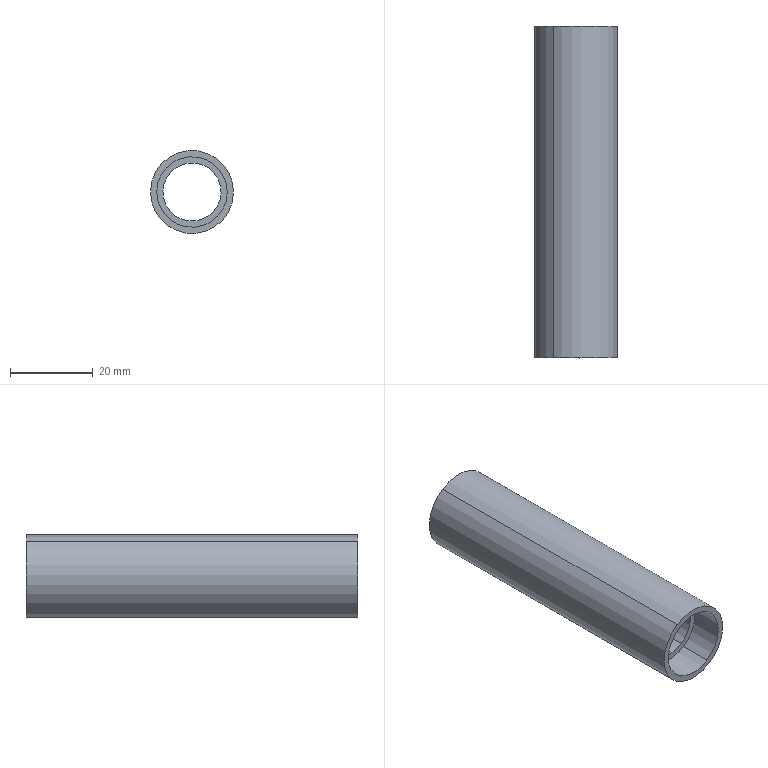Component | SolidWorks | JL001-03-06-1_JL001-03-06-002-1 | 1 solid | 12 faces | box 20 x 80 x 20 mm | volume 11649 mm3 | cylinder 8 | plane 4 | commonest cylinder face diameters 17 x4 14 x2 20 x2
build123d program:
from build123d import *


with BuildPart() as part:
    # Sketch1 → Revolve1 (revolve)
    with BuildSketch(Plane.XY, mode=Mode.PRIVATE) as revolve1_sk:
        Polygon((8.5, 0), (10, 0), (10, -80), (8.5, -80), (8.5, -72), (7, -72), (7, -8), (8.5, -8), align=None)
    revolve(revolve1_sk.sketch.rotate(Axis((0, 0, 0), (0, -1, 0)), 90), axis=Axis((0, 0, 0), (0, -1, 0)))


solid = part.part

# Placed as in the assembly
solid = solid.moved(Location((-69, 1117, 65), (0, 0, 0)))
STEP:
#1=COLOUR_RGB('',0.7922,0.8196,0.9333);
#2=FILL_AREA_STYLE_COLOUR('',#1);
#3=FILL_AREA_STYLE('',(#2));
#4=SURFACE_STYLE_FILL_AREA(#3);
#5=SURFACE_SIDE_STYLE('',(#4));
#6=SURFACE_STYLE_USAGE(.BOTH.,#5);
#7=PRESENTATION_STYLE_ASSIGNMENT((#6));
#8=CARTESIAN_POINT('',(-2.867,43.661,2.79));
#9=VERTEX_POINT('',#8);
#10=CARTESIAN_POINT('',(-2.566,43.661,2.328));
#11=VERTEX_POINT('',#10);
#12=CARTESIAN_POINT('',(-2.717,43.661,2.559));
#13=DIRECTION('',(-0.,-1.,-0.));
#14=DIRECTION('',(0.5469,0.,-0.8372));
#15=AXIS2_PLACEMENT_3D('',#12,#13,#14);
#16=CIRCLE('',#15,0.2756);
#17=EDGE_CURVE('',#9,#11,#16,.T.);
#18=ORIENTED_EDGE('',*,*,#17,.F.);
#19=CARTESIAN_POINT('',(-2.867,41.142,2.79));
#20=VERTEX_POINT('',#19);
#21=CARTESIAN_POINT('',(-2.867,40.827,2.79));
#22=DIRECTION('',(-0.,-1.,-0.));
#23=VECTOR('',#22,39.37);
#24=LINE('',#21,#23);
#25=EDGE_CURVE('',#9,#20,#24,.T.);
#26=ORIENTED_EDGE('',*,*,#25,.T.);
#27=CARTESIAN_POINT('',(-2.566,41.142,2.328));
#28=VERTEX_POINT('',#27);
#29=CARTESIAN_POINT('',(-2.717,41.142,2.559));
#30=DIRECTION('',(-0.,-1.,-0.));
#31=DIRECTION('',(0.5469,0.,-0.8372));
#32=AXIS2_PLACEMENT_3D('',#29,#30,#31);
#33=CIRCLE('',#32,0.2756);
#34=EDGE_CURVE('',#20,#28,#33,.T.);
#35=ORIENTED_EDGE('',*,*,#34,.T.);
#36=CARTESIAN_POINT('',(-2.566,40.827,2.328));
#37=DIRECTION('',(-0.,-1.,-0.));
#38=VECTOR('',#37,39.37);
#39=LINE('',#36,#38);
#40=EDGE_CURVE('',#11,#28,#39,.T.);
#41=ORIENTED_EDGE('',*,*,#40,.F.);
#42=EDGE_LOOP('',(#18,#26,#35,#41));
#43=FACE_OUTER_BOUND('',#42,.T.);
#44=CARTESIAN_POINT('',(-2.717,40.827,2.559));
#45=DIRECTION('',(-0.,-1.,-0.));
#46=DIRECTION('',(0.5469,0.,-0.8372));
#47=AXIS2_PLACEMENT_3D('',#44,#45,#46);
#48=CYLINDRICAL_SURFACE('',#47,0.2756);
#49=ADVANCED_FACE('',(#43),#48,.F.);
#50=CARTESIAN_POINT('',(-2.9,43.976,2.839));
#51=VERTEX_POINT('',#50);
#52=CARTESIAN_POINT('',(-2.534,43.976,2.279));
#53=VERTEX_POINT('',#52);
#54=CARTESIAN_POINT('',(-2.717,43.976,2.559));
#55=DIRECTION('',(-0.,-1.,-0.));
#56=DIRECTION('',(0.5469,0.,-0.8372));
#57=AXIS2_PLACEMENT_3D('',#54,#55,#56);
#58=CIRCLE('',#57,0.3346);
#59=EDGE_CURVE('',#51,#53,#58,.T.);
#60=ORIENTED_EDGE('',*,*,#59,.F.);
#61=CARTESIAN_POINT('',(-2.9,43.661,2.839));
#62=VERTEX_POINT('',#61);
#63=CARTESIAN_POINT('',(-2.9,40.827,2.839));
#64=DIRECTION('',(-0.,-1.,-0.));
#65=VECTOR('',#64,39.37);
#66=LINE('',#63,#65);
#67=EDGE_CURVE('',#51,#62,#66,.T.);
#68=ORIENTED_EDGE('',*,*,#67,.T.);
#69=CARTESIAN_POINT('',(-2.534,43.661,2.279));
#70=VERTEX_POINT('',#69);
#71=CARTESIAN_POINT('',(-2.717,43.661,2.559));
#72=DIRECTION('',(-0.,-1.,-0.));
#73=DIRECTION('',(0.5469,0.,-0.8372));
#74=AXIS2_PLACEMENT_3D('',#71,#72,#73);
#75=CIRCLE('',#74,0.3346);
#76=EDGE_CURVE('',#62,#70,#75,.T.);
#77=ORIENTED_EDGE('',*,*,#76,.T.);
#78=CARTESIAN_POINT('',(-2.534,40.827,2.279));
#79=DIRECTION('',(-0.,-1.,-0.));
#80=VECTOR('',#79,39.37);
#81=LINE('',#78,#80);
#82=EDGE_CURVE('',#53,#70,#81,.T.);
#83=ORIENTED_EDGE('',*,*,#82,.F.);
#84=EDGE_LOOP('',(#60,#68,#77,#83));
#85=FACE_OUTER_BOUND('',#84,.T.);
#86=CARTESIAN_POINT('',(-2.717,40.827,2.559));
#87=DIRECTION('',(-0.,-1.,-0.));
#88=DIRECTION('',(0.5469,0.,-0.8372));
#89=AXIS2_PLACEMENT_3D('',#86,#87,#88);
#90=CYLINDRICAL_SURFACE('',#89,0.3346);
#91=ADVANCED_FACE('',(#85),#90,.F.);
#92=CARTESIAN_POINT('',(-2.501,43.976,2.229));
#93=VERTEX_POINT('',#92);
#94=CARTESIAN_POINT('',(-2.932,43.976,2.889));
#95=VERTEX_POINT('',#94);
#96=CARTESIAN_POINT('',(-2.717,43.976,2.559));
#97=DIRECTION('',(-0.,-1.,-0.));
#98=DIRECTION('',(0.5469,0.,-0.8372));
#99=AXIS2_PLACEMENT_3D('',#96,#97,#98);
#100=CIRCLE('',#99,0.3937);
#101=EDGE_CURVE('',#93,#95,#100,.T.);
#102=ORIENTED_EDGE('',*,*,#101,.T.);
#103=CARTESIAN_POINT('',(-2.932,40.827,2.889));
#104=VERTEX_POINT('',#103);
#105=CARTESIAN_POINT('',(-2.932,40.827,2.889));
#106=DIRECTION('',(-0.,-1.,-0.));
#107=VECTOR('',#106,39.37);
#108=LINE('',#105,#107);
#109=EDGE_CURVE('',#95,#104,#108,.T.);
#110=ORIENTED_EDGE('',*,*,#109,.T.);
#111=CARTESIAN_POINT('',(-2.501,40.827,2.229));
#112=VERTEX_POINT('',#111);
#113=CARTESIAN_POINT('',(-2.717,40.827,2.559));
#114=DIRECTION('',(-0.,-1.,-0.));
#115=DIRECTION('',(0.5469,0.,-0.8372));
#116=AXIS2_PLACEMENT_3D('',#113,#114,#115);
#117=CIRCLE('',#116,0.3937);
#118=EDGE_CURVE('',#112,#104,#117,.T.);
#119=ORIENTED_EDGE('',*,*,#118,.F.);
#120=CARTESIAN_POINT('',(-2.501,40.827,2.229));
#121=DIRECTION('',(-0.,-1.,-0.));
#122=VECTOR('',#121,39.37);
#123=LINE('',#120,#122);
#124=EDGE_CURVE('',#93,#112,#123,.T.);
#125=ORIENTED_EDGE('',*,*,#124,.F.);
#126=EDGE_LOOP('',(#102,#110,#119,#125));
#127=FACE_OUTER_BOUND('',#126,.T.);
#128=CARTESIAN_POINT('',(-2.717,40.827,2.559));
#129=DIRECTION('',(-0.,-1.,-0.));
#130=DIRECTION('',(0.5469,0.,-0.8372));
#131=AXIS2_PLACEMENT_3D('',#128,#129,#130);
#132=CYLINDRICAL_SURFACE('',#131,0.3937);
#133=ADVANCED_FACE('',(#127),#132,.T.);
#134=CARTESIAN_POINT('',(-2.9,41.142,2.839));
#135=VERTEX_POINT('',#134);
#136=CARTESIAN_POINT('',(-2.534,41.142,2.279));
#137=VERTEX_POINT('',#136);
#138=CARTESIAN_POINT('',(-2.717,41.142,2.559));
#139=DIRECTION('',(-0.,-1.,-0.));
#140=DIRECTION('',(0.5469,0.,-0.8372));
#141=AXIS2_PLACEMENT_3D('',#138,#139,#140);
#142=CIRCLE('',#141,0.3346);
#143=EDGE_CURVE('',#135,#137,#142,.T.);
#144=ORIENTED_EDGE('',*,*,#143,.F.);
#145=CARTESIAN_POINT('',(-2.9,40.827,2.839));
#146=VERTEX_POINT('',#145);
#147=CARTESIAN_POINT('',(-2.9,40.827,2.839));
#148=DIRECTION('',(-0.,-1.,-0.));
#149=VECTOR('',#148,39.37);
#150=LINE('',#147,#149);
#151=EDGE_CURVE('',#135,#146,#150,.T.);
#152=ORIENTED_EDGE('',*,*,#151,.T.);
#153=CARTESIAN_POINT('',(-2.534,40.827,2.279));
#154=VERTEX_POINT('',#153);
#155=CARTESIAN_POINT('',(-2.717,40.827,2.559));
#156=DIRECTION('',(-0.,-1.,-0.));
#157=DIRECTION('',(0.5469,0.,-0.8372));
#158=AXIS2_PLACEMENT_3D('',#155,#156,#157);
#159=CIRCLE('',#158,0.3346);
#160=EDGE_CURVE('',#146,#154,#159,.T.);
#161=ORIENTED_EDGE('',*,*,#160,.T.);
#162=CARTESIAN_POINT('',(-2.534,40.827,2.279));
#163=DIRECTION('',(-0.,-1.,-0.));
#164=VECTOR('',#163,39.37);
#165=LINE('',#162,#164);
#166=EDGE_CURVE('',#137,#154,#165,.T.);
#167=ORIENTED_EDGE('',*,*,#166,.F.);
#168=EDGE_LOOP('',(#144,#152,#161,#167));
#169=FACE_OUTER_BOUND('',#168,.T.);
#170=CARTESIAN_POINT('',(-2.717,40.827,2.559));
#171=DIRECTION('',(-0.,-1.,-0.));
#172=DIRECTION('',(0.5469,0.,-0.8372));
#173=AXIS2_PLACEMENT_3D('',#170,#171,#172);
#174=CYLINDRICAL_SURFACE('',#173,0.3346);
#175=ADVANCED_FACE('',(#169),#174,.F.);
#176=ORIENTED_EDGE('',*,*,#151,.F.);
#177=CARTESIAN_POINT('',(-2.717,41.142,2.559));
#178=DIRECTION('',(-0.,-1.,-0.));
#179=DIRECTION('',(0.5469,0.,-0.8372));
#180=AXIS2_PLACEMENT_3D('',#177,#178,#179);
#181=CIRCLE('',#180,0.3346);
#182=EDGE_CURVE('',#137,#135,#181,.T.);
#183=ORIENTED_EDGE('',*,*,#182,.F.);
#184=ORIENTED_EDGE('',*,*,#166,.T.);
#185=CARTESIAN_POINT('',(-2.717,40.827,2.559));
#186=DIRECTION('',(-0.,-1.,-0.));
#187=DIRECTION('',(0.5469,0.,-0.8372));
#188=AXIS2_PLACEMENT_3D('',#185,#186,#187);
#189=CIRCLE('',#188,0.3346);
#190=EDGE_CURVE('',#154,#146,#189,.T.);
#191=ORIENTED_EDGE('',*,*,#190,.T.);
#192=EDGE_LOOP('',(#176,#183,#184,#191));
#193=FACE_OUTER_BOUND('',#192,.T.);
#194=CARTESIAN_POINT('',(-2.717,40.827,2.559));
#195=DIRECTION('',(-0.,-1.,-0.));
#196=DIRECTION('',(0.5469,0.,-0.8372));
#197=AXIS2_PLACEMENT_3D('',#194,#195,#196);
#198=CYLINDRICAL_SURFACE('',#197,0.3346);
#199=ADVANCED_FACE('',(#193),#198,.F.);
#200=ORIENTED_EDGE('',*,*,#190,.F.);
#201=ORIENTED_EDGE('',*,*,#160,.F.);
#202=EDGE_LOOP('',(#200,#201));
#203=FACE_BOUND('',#202,.T.);
#204=ORIENTED_EDGE('',*,*,#118,.T.);
#205=CARTESIAN_POINT('',(-2.717,40.827,2.559));
#206=DIRECTION('',(-0.,-1.,-0.));
#207=DIRECTION('',(0.5469,0.,-0.8372));
#208=AXIS2_PLACEMENT_3D('',#205,#206,#207);
#209=CIRCLE('',#208,0.3937);
#210=EDGE_CURVE('',#104,#112,#209,.T.);
#211=ORIENTED_EDGE('',*,*,#210,.T.);
#212=EDGE_LOOP('',(#204,#211));
#213=FACE_OUTER_BOUND('',#212,.T.);
#214=CARTESIAN_POINT('',(-2.436,40.827,2.742));
#215=DIRECTION('',(-0.,1.,0.));
#216=DIRECTION('',(-0.5469,-0.,0.8372));
#217=AXIS2_PLACEMENT_3D('',#214,#215,#216);
#218=PLANE('',#217);
#219=ADVANCED_FACE('',(#203,#213),#218,.F.);
#220=ORIENTED_EDGE('',*,*,#109,.F.);
#221=CARTESIAN_POINT('',(-2.717,43.976,2.559));
#222=DIRECTION('',(-0.,-1.,-0.));
#223=DIRECTION('',(0.5469,0.,-0.8372));
#224=AXIS2_PLACEMENT_3D('',#221,#222,#223);
#225=CIRCLE('',#224,0.3937);
#226=EDGE_CURVE('',#95,#93,#225,.T.);
#227=ORIENTED_EDGE('',*,*,#226,.T.);
#228=ORIENTED_EDGE('',*,*,#124,.T.);
#229=ORIENTED_EDGE('',*,*,#210,.F.);
#230=EDGE_LOOP('',(#220,#227,#228,#229));
#231=FACE_OUTER_BOUND('',#230,.T.);
#232=CARTESIAN_POINT('',(-2.717,40.827,2.559));
#233=DIRECTION('',(-0.,-1.,-0.));
#234=DIRECTION('',(0.5469,0.,-0.8372));
#235=AXIS2_PLACEMENT_3D('',#232,#233,#234);
#236=CYLINDRICAL_SURFACE('',#235,0.3937);
#237=ADVANCED_FACE('',(#231),#236,.T.);
#238=ORIENTED_EDGE('',*,*,#101,.F.);
#239=ORIENTED_EDGE('',*,*,#226,.F.);
#240=EDGE_LOOP('',(#238,#239));
#241=FACE_OUTER_BOUND('',#240,.T.);
#242=CARTESIAN_POINT('',(-2.717,43.976,2.559));
#243=DIRECTION('',(-0.,-1.,-0.));
#244=DIRECTION('',(0.5469,0.,-0.8372));
#245=AXIS2_PLACEMENT_3D('',#242,#243,#244);
#246=CIRCLE('',#245,0.3346);
#247=EDGE_CURVE('',#53,#51,#246,.T.);
#248=ORIENTED_EDGE('',*,*,#247,.T.);
#249=ORIENTED_EDGE('',*,*,#59,.T.);
#250=EDGE_LOOP('',(#248,#249));
#251=FACE_BOUND('',#250,.T.);
#252=CARTESIAN_POINT('',(-2.387,43.976,2.774));
#253=DIRECTION('',(0.,-1.,-0.));
#254=DIRECTION('',(0.5469,0.,-0.8372));
#255=AXIS2_PLACEMENT_3D('',#252,#253,#254);
#256=PLANE('',#255);
#257=ADVANCED_FACE('',(#241,#251),#256,.F.);
#258=ORIENTED_EDGE('',*,*,#67,.F.);
#259=ORIENTED_EDGE('',*,*,#247,.F.);
#260=ORIENTED_EDGE('',*,*,#82,.T.);
#261=CARTESIAN_POINT('',(-2.717,43.661,2.559));
#262=DIRECTION('',(-0.,-1.,-0.));
#263=DIRECTION('',(0.5469,0.,-0.8372));
#264=AXIS2_PLACEMENT_3D('',#261,#262,#263);
#265=CIRCLE('',#264,0.3346);
#266=EDGE_CURVE('',#70,#62,#265,.T.);
#267=ORIENTED_EDGE('',*,*,#266,.T.);
#268=EDGE_LOOP('',(#258,#259,#260,#267));
#269=FACE_OUTER_BOUND('',#268,.T.);
#270=CARTESIAN_POINT('',(-2.717,40.827,2.559));
#271=DIRECTION('',(-0.,-1.,-0.));
#272=DIRECTION('',(0.5469,0.,-0.8372));
#273=AXIS2_PLACEMENT_3D('',#270,#271,#272);
#274=CYLINDRICAL_SURFACE('',#273,0.3346);
#275=ADVANCED_FACE('',(#269),#274,.F.);
#276=ORIENTED_EDGE('',*,*,#266,.F.);
#277=ORIENTED_EDGE('',*,*,#76,.F.);
#278=EDGE_LOOP('',(#276,#277));
#279=FACE_OUTER_BOUND('',#278,.T.);
#280=CARTESIAN_POINT('',(-2.717,43.661,2.559));
#281=DIRECTION('',(-0.,-1.,-0.));
#282=DIRECTION('',(0.5469,0.,-0.8372));
#283=AXIS2_PLACEMENT_3D('',#280,#281,#282);
#284=CIRCLE('',#283,0.2756);
#285=EDGE_CURVE('',#11,#9,#284,.T.);
#286=ORIENTED_EDGE('',*,*,#285,.T.);
#287=ORIENTED_EDGE('',*,*,#17,.T.);
#288=EDGE_LOOP('',(#286,#287));
#289=FACE_BOUND('',#288,.T.);
#290=CARTESIAN_POINT('',(-2.436,43.661,2.742));
#291=DIRECTION('',(0.,-1.,-0.));
#292=DIRECTION('',(0.5469,0.,-0.8372));
#293=AXIS2_PLACEMENT_3D('',#290,#291,#292);
#294=PLANE('',#293);
#295=ADVANCED_FACE('',(#279,#289),#294,.F.);
#296=ORIENTED_EDGE('',*,*,#25,.F.);
#297=ORIENTED_EDGE('',*,*,#285,.F.);
#298=ORIENTED_EDGE('',*,*,#40,.T.);
#299=CARTESIAN_POINT('',(-2.717,41.142,2.559));
#300=DIRECTION('',(-0.,-1.,-0.));
#301=DIRECTION('',(0.5469,0.,-0.8372));
#302=AXIS2_PLACEMENT_3D('',#299,#300,#301);
#303=CIRCLE('',#302,0.2756);
#304=EDGE_CURVE('',#28,#20,#303,.T.);
#305=ORIENTED_EDGE('',*,*,#304,.T.);
#306=EDGE_LOOP('',(#296,#297,#298,#305));
#307=FACE_OUTER_BOUND('',#306,.T.);
#308=CARTESIAN_POINT('',(-2.717,40.827,2.559));
#309=DIRECTION('',(-0.,-1.,-0.));
#310=DIRECTION('',(0.5469,0.,-0.8372));
#311=AXIS2_PLACEMENT_3D('',#308,#309,#310);
#312=CYLINDRICAL_SURFACE('',#311,0.2756);
#313=ADVANCED_FACE('',(#307),#312,.F.);
#314=ORIENTED_EDGE('',*,*,#304,.F.);
#315=ORIENTED_EDGE('',*,*,#34,.F.);
#316=EDGE_LOOP('',(#314,#315));
#317=FACE_BOUND('',#316,.T.);
#318=ORIENTED_EDGE('',*,*,#182,.T.);
#319=ORIENTED_EDGE('',*,*,#143,.T.);
#320=EDGE_LOOP('',(#318,#319));
#321=FACE_OUTER_BOUND('',#320,.T.);
#322=CARTESIAN_POINT('',(-2.486,41.142,2.71));
#323=DIRECTION('',(-0.,1.,0.));
#324=DIRECTION('',(-0.5469,-0.,0.8372));
#325=AXIS2_PLACEMENT_3D('',#322,#323,#324);
#326=PLANE('',#325);
#327=ADVANCED_FACE('',(#317,#321),#326,.F.);
#328=CLOSED_SHELL('',(#49,#91,#133,#175,#199,#219,#237,#257,#275,#295,#313,#327));
#329=MANIFOLD_SOLID_BREP('',#328);
#330=STYLED_ITEM('',(#7),#329);
#331=(LENGTH_UNIT()NAMED_UNIT(*)SI_UNIT($,.METRE.));
#332=LENGTH_MEASURE_WITH_UNIT(LENGTH_MEASURE(0.0254),#331);
#333=DIMENSIONAL_EXPONENTS(1.,0.,0.,0.,0.,0.,0.);
#334=(CONVERSION_BASED_UNIT('',#332)LENGTH_UNIT()NAMED_UNIT(#333));
#335=UNCERTAINTY_MEASURE_WITH_UNIT(LENGTH_MEASURE(0.00001),#334,'','');
#336=(NAMED_UNIT(*)PLANE_ANGLE_UNIT()SI_UNIT($,.RADIAN.));
#337=(NAMED_UNIT(*)SI_UNIT($,.STERADIAN.)SOLID_ANGLE_UNIT());
#338=(GEOMETRIC_REPRESENTATION_CONTEXT(3)GLOBAL_UNCERTAINTY_ASSIGNED_CONTEXT((#335))GLOBAL_UNIT_ASSIGNED_CONTEXT((#334,#336,#337))REPRESENTATION_CONTEXT('',''));
#339=MECHANICAL_DESIGN_GEOMETRIC_PRESENTATION_REPRESENTATION('',(#330),#338);
#340=CARTESIAN_POINT('',(0.,0.,0.));
#341=DIRECTION('',(0.,0.,1.));
#342=DIRECTION('',(1.,0.,0.));
#343=AXIS2_PLACEMENT_3D('',#340,#341,#342);
#344=(LENGTH_UNIT()NAMED_UNIT(*)SI_UNIT($,.METRE.));
#345=LENGTH_MEASURE_WITH_UNIT(LENGTH_MEASURE(0.0254),#344);
#346=DIMENSIONAL_EXPONENTS(1.,0.,0.,0.,0.,0.,0.);
#347=(CONVERSION_BASED_UNIT('',#345)LENGTH_UNIT()NAMED_UNIT(#346));
#348=UNCERTAINTY_MEASURE_WITH_UNIT(LENGTH_MEASURE(0.00001),#347,'','');
#349=(NAMED_UNIT(*)PLANE_ANGLE_UNIT()SI_UNIT($,.RADIAN.));
#350=(NAMED_UNIT(*)SI_UNIT($,.STERADIAN.)SOLID_ANGLE_UNIT());
#351=(GEOMETRIC_REPRESENTATION_CONTEXT(3)GLOBAL_UNCERTAINTY_ASSIGNED_CONTEXT((#348))GLOBAL_UNIT_ASSIGNED_CONTEXT((#347,#349,#350))REPRESENTATION_CONTEXT('',''));
#352=ADVANCED_BREP_SHAPE_REPRESENTATION('',(#329,#343),#351);
#353=PRESENTATION_LAYER_ASSIGNMENT('','',(#330));